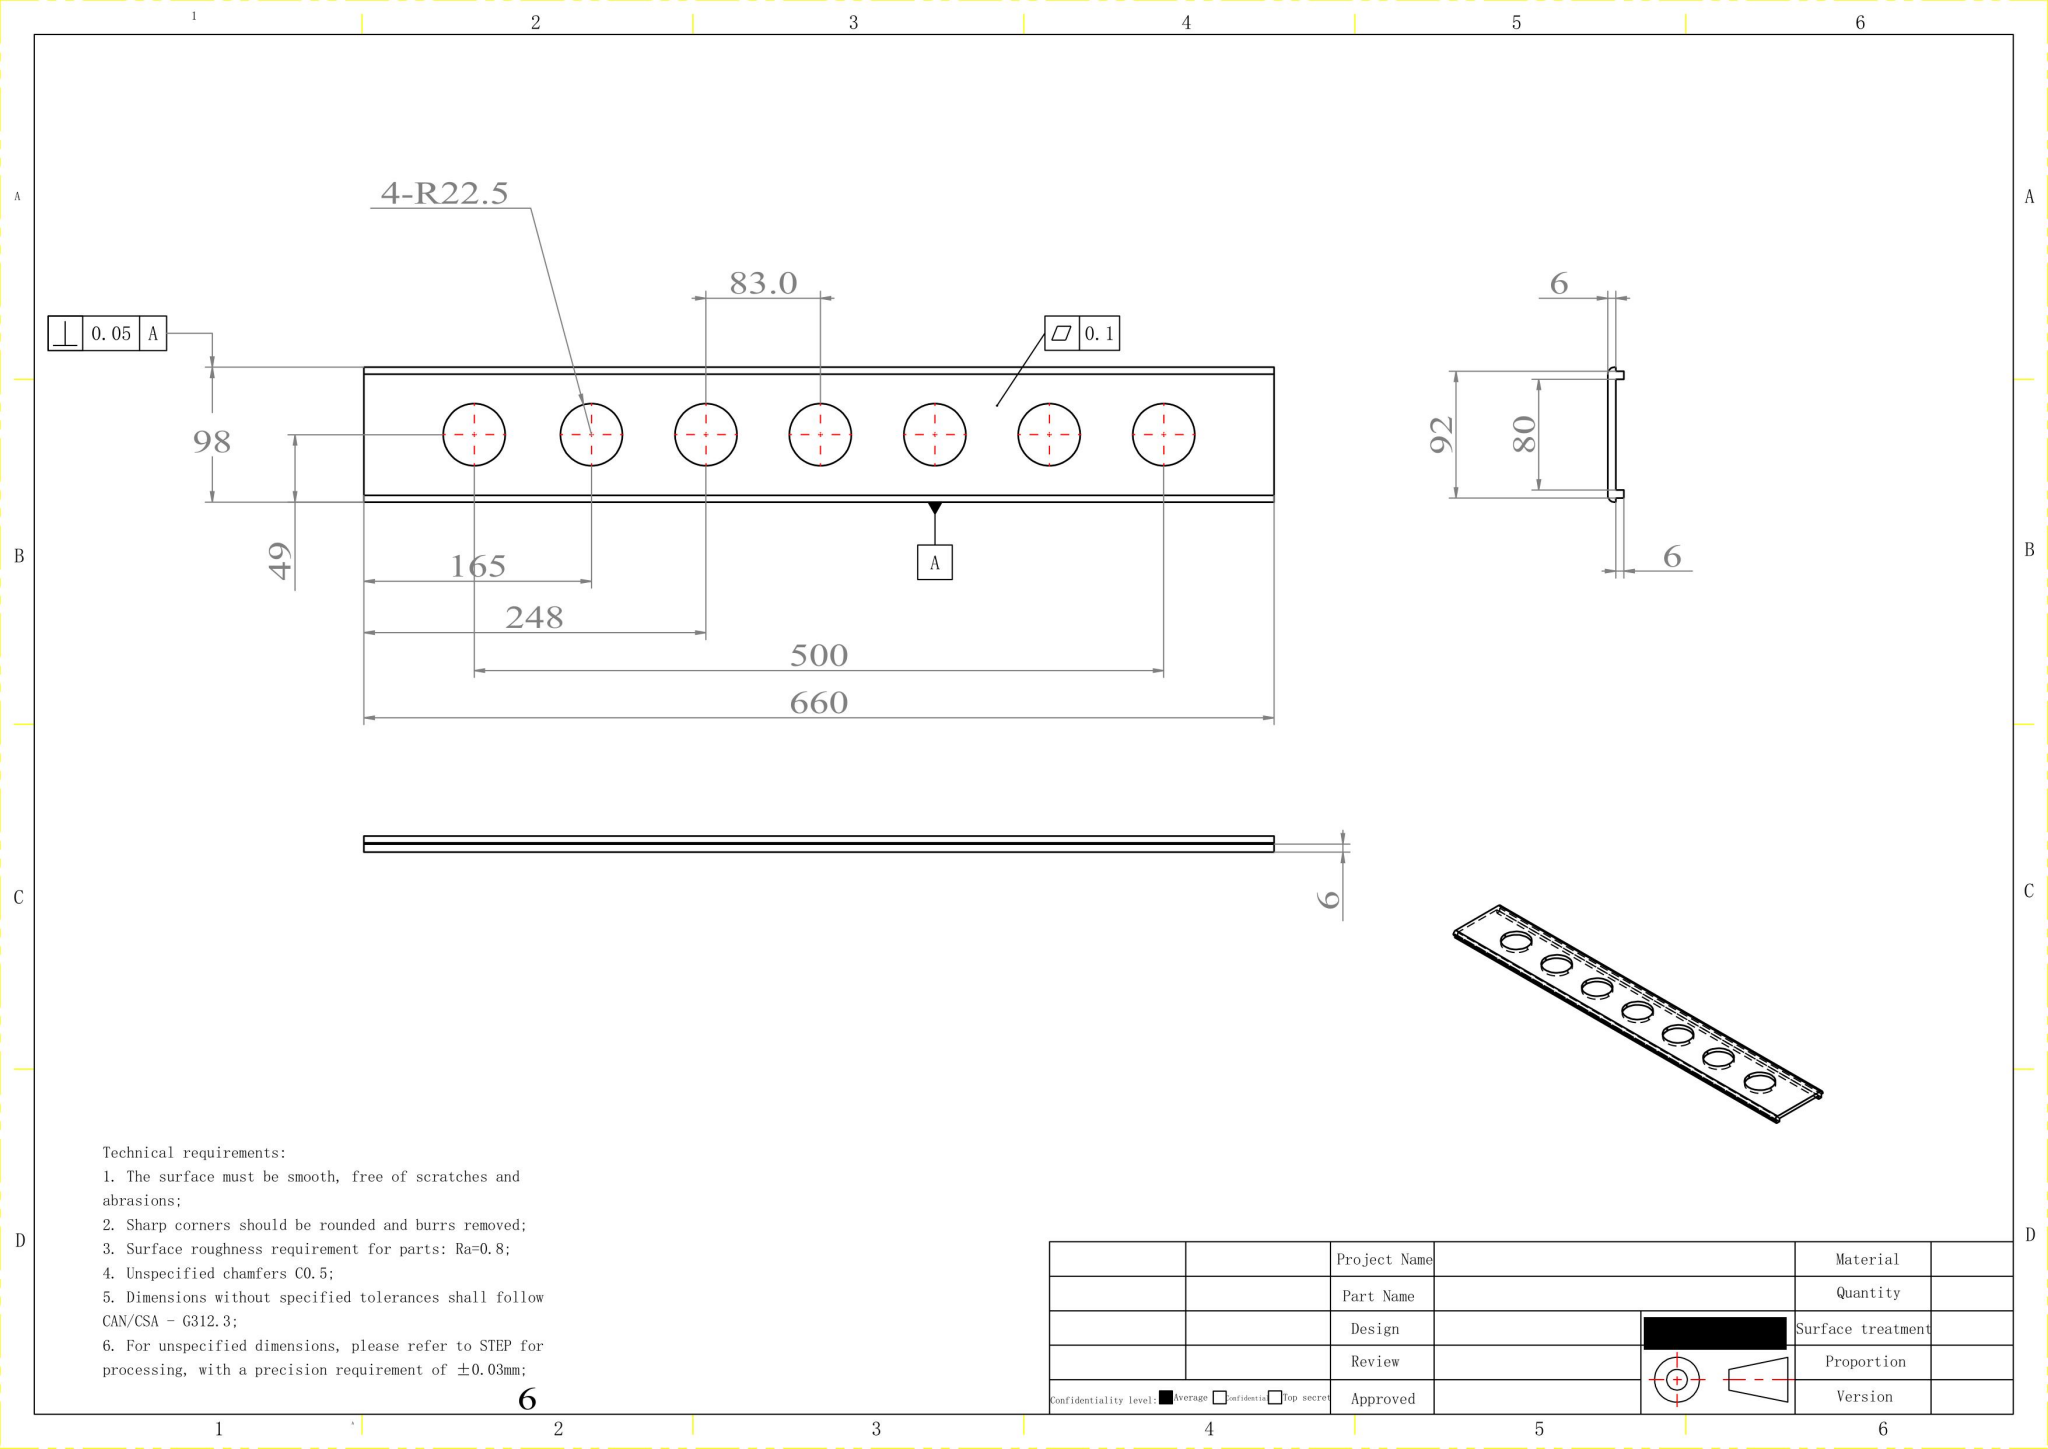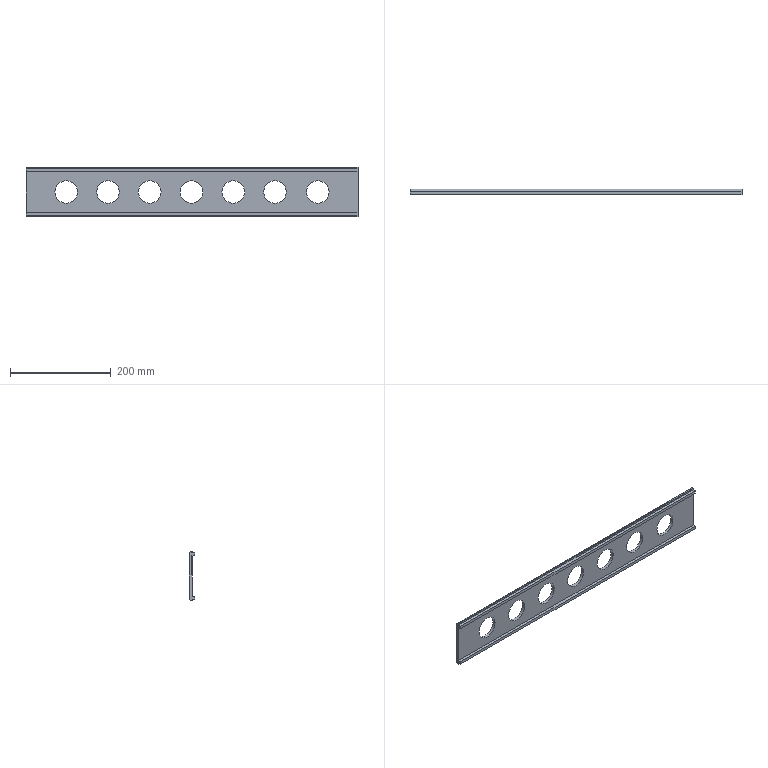Part | SolidWorks | mm | 1 solid | 30 faces | box 660 x 11.68 x 97.82 mm | volume 349958 mm3 | cylinder 16 | plane 14 | commonest cylinder face diameters 45 x14 10 x2
STEP:
#1=CARTESIAN_POINT('',(-165.31,-9.,-30.01));
#2=VERTEX_POINT('',#1);
#3=CARTESIAN_POINT('',(-825.31,-9.,-30.01));
#4=VERTEX_POINT('',#3);
#5=CARTESIAN_POINT('',(-165.31,-9.,-30.01));
#6=DIRECTION('',(-1.,0.,0.));
#7=VECTOR('',#6,1000.);
#8=LINE('',#5,#7);
#9=EDGE_CURVE('',#2,#4,#8,.T.);
#10=ORIENTED_EDGE('',*,*,#9,.F.);
#11=CARTESIAN_POINT('',(-165.31,-9.84,-30.01));
#12=VERTEX_POINT('',#11);
#13=CARTESIAN_POINT('',(-165.31,-9.84,-30.01));
#14=DIRECTION('',(0.,1.,-0.));
#15=VECTOR('',#14,1000.);
#16=LINE('',#13,#15);
#17=EDGE_CURVE('',#12,#2,#16,.T.);
#18=ORIENTED_EDGE('',*,*,#17,.F.);
#19=CARTESIAN_POINT('',(-825.31,-9.84,-30.01));
#20=VERTEX_POINT('',#19);
#21=CARTESIAN_POINT('',(-825.31,-9.84,-30.01));
#22=DIRECTION('',(1.,0.,0.));
#23=VECTOR('',#22,1000.);
#24=LINE('',#21,#23);
#25=EDGE_CURVE('',#20,#12,#24,.T.);
#26=ORIENTED_EDGE('',*,*,#25,.F.);
#27=CARTESIAN_POINT('',(-825.31,-9.,-30.01));
#28=DIRECTION('',(0.,-1.,0.));
#29=VECTOR('',#28,1000.);
#30=LINE('',#27,#29);
#31=EDGE_CURVE('',#4,#20,#30,.T.);
#32=ORIENTED_EDGE('',*,*,#31,.F.);
#33=EDGE_LOOP('',(#10,#18,#26,#32));
#34=FACE_OUTER_BOUND('',#33,.T.);
#35=CARTESIAN_POINT('',(-495.31,-9.84,-30.01));
#36=DIRECTION('',(0.,0.,-1.));
#37=DIRECTION('',(0.,-1.,0.));
#38=AXIS2_PLACEMENT_3D('',#35,#36,#37);
#39=PLANE('',#38);
#40=ADVANCED_FACE('',(#34),#39,.T.);
#41=CARTESIAN_POINT('',(-825.31,-4.,62.81));
#42=VERTEX_POINT('',#41);
#43=CARTESIAN_POINT('',(-825.31,-9.,67.81));
#44=VERTEX_POINT('',#43);
#45=CARTESIAN_POINT('',(-825.31,-9.,62.81));
#46=DIRECTION('',(1.,0.,0.));
#47=DIRECTION('',(-0.,1.,-0.));
#48=AXIS2_PLACEMENT_3D('',#45,#46,#47);
#49=CIRCLE('',#48,5.);
#50=EDGE_CURVE('',#42,#44,#49,.T.);
#51=ORIENTED_EDGE('',*,*,#50,.F.);
#52=CARTESIAN_POINT('',(-825.31,-4.,-25.01));
#53=VERTEX_POINT('',#52);
#54=CARTESIAN_POINT('',(-825.31,-4.,-25.01));
#55=DIRECTION('',(0.,0.,1.));
#56=VECTOR('',#55,1000.);
#57=LINE('',#54,#56);
#58=EDGE_CURVE('',#53,#42,#57,.T.);
#59=ORIENTED_EDGE('',*,*,#58,.F.);
#60=CARTESIAN_POINT('',(-825.31,-9.,-25.01));
#61=DIRECTION('',(1.,0.,-0.));
#62=DIRECTION('',(-0.,0.,-1.));
#63=AXIS2_PLACEMENT_3D('',#60,#61,#62);
#64=CIRCLE('',#63,5.);
#65=EDGE_CURVE('',#4,#53,#64,.T.);
#66=ORIENTED_EDGE('',*,*,#65,.F.);
#67=ORIENTED_EDGE('',*,*,#31,.T.);
#68=CARTESIAN_POINT('',(-825.31,-9.84,-27.09));
#69=VERTEX_POINT('',#68);
#70=CARTESIAN_POINT('',(-825.31,-9.84,-27.09));
#71=DIRECTION('',(0.,0.,-1.));
#72=VECTOR('',#71,1000.);
#73=LINE('',#70,#72);
#74=EDGE_CURVE('',#69,#20,#73,.T.);
#75=ORIENTED_EDGE('',*,*,#74,.F.);
#76=CARTESIAN_POINT('',(-825.31,-15.68,-27.09));
#77=VERTEX_POINT('',#76);
#78=CARTESIAN_POINT('',(-825.31,-15.68,-27.09));
#79=DIRECTION('',(0.,1.,0.));
#80=VECTOR('',#79,1000.);
#81=LINE('',#78,#80);
#82=EDGE_CURVE('',#77,#69,#81,.T.);
#83=ORIENTED_EDGE('',*,*,#82,.F.);
#84=CARTESIAN_POINT('',(-825.31,-15.68,-21.25));
#85=VERTEX_POINT('',#84);
#86=CARTESIAN_POINT('',(-825.31,-15.68,-21.25));
#87=DIRECTION('',(0.,0.,-1.));
#88=VECTOR('',#87,1000.);
#89=LINE('',#86,#88);
#90=EDGE_CURVE('',#85,#77,#89,.T.);
#91=ORIENTED_EDGE('',*,*,#90,.F.);
#92=CARTESIAN_POINT('',(-825.31,-9.84,-21.25));
#93=VERTEX_POINT('',#92);
#94=CARTESIAN_POINT('',(-825.31,-9.84,-21.25));
#95=DIRECTION('',(0.,-1.,0.));
#96=VECTOR('',#95,1000.);
#97=LINE('',#94,#96);
#98=EDGE_CURVE('',#93,#85,#97,.T.);
#99=ORIENTED_EDGE('',*,*,#98,.F.);
#100=CARTESIAN_POINT('',(-825.31,-9.84,59.05));
#101=VERTEX_POINT('',#100);
#102=CARTESIAN_POINT('',(-825.31,-9.84,59.05));
#103=DIRECTION('',(0.,0.,-1.));
#104=VECTOR('',#103,1000.);
#105=LINE('',#102,#104);
#106=EDGE_CURVE('',#101,#93,#105,.T.);
#107=ORIENTED_EDGE('',*,*,#106,.F.);
#108=CARTESIAN_POINT('',(-825.31,-15.68,59.05));
#109=VERTEX_POINT('',#108);
#110=CARTESIAN_POINT('',(-825.31,-15.68,59.05));
#111=DIRECTION('',(0.,1.,0.));
#112=VECTOR('',#111,1000.);
#113=LINE('',#110,#112);
#114=EDGE_CURVE('',#109,#101,#113,.T.);
#115=ORIENTED_EDGE('',*,*,#114,.F.);
#116=CARTESIAN_POINT('',(-825.31,-15.68,64.89));
#117=VERTEX_POINT('',#116);
#118=CARTESIAN_POINT('',(-825.31,-15.68,64.89));
#119=DIRECTION('',(0.,0.,-1.));
#120=VECTOR('',#119,1000.);
#121=LINE('',#118,#120);
#122=EDGE_CURVE('',#117,#109,#121,.T.);
#123=ORIENTED_EDGE('',*,*,#122,.F.);
#124=CARTESIAN_POINT('',(-825.31,-9.84,64.89));
#125=VERTEX_POINT('',#124);
#126=CARTESIAN_POINT('',(-825.31,-9.84,64.89));
#127=DIRECTION('',(0.,-1.,0.));
#128=VECTOR('',#127,1000.);
#129=LINE('',#126,#128);
#130=EDGE_CURVE('',#125,#117,#129,.T.);
#131=ORIENTED_EDGE('',*,*,#130,.F.);
#132=CARTESIAN_POINT('',(-825.31,-9.84,67.81));
#133=VERTEX_POINT('',#132);
#134=CARTESIAN_POINT('',(-825.31,-9.84,67.81));
#135=DIRECTION('',(0.,0.,-1.));
#136=VECTOR('',#135,1000.);
#137=LINE('',#134,#136);
#138=EDGE_CURVE('',#133,#125,#137,.T.);
#139=ORIENTED_EDGE('',*,*,#138,.F.);
#140=CARTESIAN_POINT('',(-825.31,-9.,67.81));
#141=DIRECTION('',(0.,-1.,0.));
#142=VECTOR('',#141,1000.);
#143=LINE('',#140,#142);
#144=EDGE_CURVE('',#44,#133,#143,.T.);
#145=ORIENTED_EDGE('',*,*,#144,.F.);
#146=EDGE_LOOP('',(#51,#59,#66,#67,#75,#83,#91,#99,#107,#115,#123,#131,#139,#145));
#147=FACE_OUTER_BOUND('',#146,.T.);
#148=CARTESIAN_POINT('',(-825.31,-4.,-35.85));
#149=DIRECTION('',(-1.,0.,0.));
#150=DIRECTION('',(0.,0.,1.));
#151=AXIS2_PLACEMENT_3D('',#148,#149,#150);
#152=PLANE('',#151);
#153=ADVANCED_FACE('',(#147),#152,.T.);
#154=CARTESIAN_POINT('',(-165.31,-9.84,-21.25));
#155=VERTEX_POINT('',#154);
#156=CARTESIAN_POINT('',(-165.31,-15.68,-21.25));
#157=VERTEX_POINT('',#156);
#158=CARTESIAN_POINT('',(-165.31,-9.84,-21.25));
#159=DIRECTION('',(0.,-1.,0.));
#160=VECTOR('',#159,1000.);
#161=LINE('',#158,#160);
#162=EDGE_CURVE('',#155,#157,#161,.T.);
#163=ORIENTED_EDGE('',*,*,#162,.F.);
#164=CARTESIAN_POINT('',(-825.31,-9.84,-21.25));
#165=DIRECTION('',(1.,0.,0.));
#166=VECTOR('',#165,1000.);
#167=LINE('',#164,#166);
#168=EDGE_CURVE('',#93,#155,#167,.T.);
#169=ORIENTED_EDGE('',*,*,#168,.F.);
#170=ORIENTED_EDGE('',*,*,#98,.T.);
#171=CARTESIAN_POINT('',(-165.31,-15.68,-21.25));
#172=DIRECTION('',(-1.,0.,0.));
#173=VECTOR('',#172,1000.);
#174=LINE('',#171,#173);
#175=EDGE_CURVE('',#157,#85,#174,.T.);
#176=ORIENTED_EDGE('',*,*,#175,.F.);
#177=EDGE_LOOP('',(#163,#169,#170,#176));
#178=FACE_OUTER_BOUND('',#177,.T.);
#179=CARTESIAN_POINT('',(-825.31,-9.84,-21.25));
#180=DIRECTION('',(0.,0.,1.));
#181=DIRECTION('',(0.,-1.,0.));
#182=AXIS2_PLACEMENT_3D('',#179,#180,#181);
#183=PLANE('',#182);
#184=ADVANCED_FACE('',(#178),#183,.T.);
#185=CARTESIAN_POINT('',(-165.31,-9.84,-27.09));
#186=VERTEX_POINT('',#185);
#187=CARTESIAN_POINT('',(-165.31,-9.84,-27.09));
#188=DIRECTION('',(0.,0.,-1.));
#189=VECTOR('',#188,1000.);
#190=LINE('',#187,#189);
#191=EDGE_CURVE('',#186,#12,#190,.T.);
#192=ORIENTED_EDGE('',*,*,#191,.F.);
#193=CARTESIAN_POINT('',(-825.31,-9.84,-27.09));
#194=DIRECTION('',(1.,0.,0.));
#195=VECTOR('',#194,1000.);
#196=LINE('',#193,#195);
#197=EDGE_CURVE('',#69,#186,#196,.T.);
#198=ORIENTED_EDGE('',*,*,#197,.F.);
#199=ORIENTED_EDGE('',*,*,#74,.T.);
#200=ORIENTED_EDGE('',*,*,#25,.T.);
#201=EDGE_LOOP('',(#192,#198,#199,#200));
#202=FACE_OUTER_BOUND('',#201,.T.);
#203=CARTESIAN_POINT('',(-825.31,-9.84,-27.09));
#204=DIRECTION('',(0.,-1.,0.));
#205=DIRECTION('',(0.,0.,-1.));
#206=AXIS2_PLACEMENT_3D('',#203,#204,#205);
#207=PLANE('',#206);
#208=ADVANCED_FACE('',(#202),#207,.T.);
#209=CARTESIAN_POINT('',(-165.31,-15.68,-27.09));
#210=VERTEX_POINT('',#209);
#211=CARTESIAN_POINT('',(-165.31,-15.68,-27.09));
#212=DIRECTION('',(0.,1.,0.));
#213=VECTOR('',#212,1000.);
#214=LINE('',#211,#213);
#215=EDGE_CURVE('',#210,#186,#214,.T.);
#216=ORIENTED_EDGE('',*,*,#215,.F.);
#217=CARTESIAN_POINT('',(-825.31,-15.68,-27.09));
#218=DIRECTION('',(1.,0.,0.));
#219=VECTOR('',#218,1000.);
#220=LINE('',#217,#219);
#221=EDGE_CURVE('',#77,#210,#220,.T.);
#222=ORIENTED_EDGE('',*,*,#221,.F.);
#223=ORIENTED_EDGE('',*,*,#82,.T.);
#224=ORIENTED_EDGE('',*,*,#197,.T.);
#225=EDGE_LOOP('',(#216,#222,#223,#224));
#226=FACE_OUTER_BOUND('',#225,.T.);
#227=CARTESIAN_POINT('',(-825.31,-9.84,-27.09));
#228=DIRECTION('',(0.,0.,-1.));
#229=DIRECTION('',(0.,-1.,0.));
#230=AXIS2_PLACEMENT_3D('',#227,#228,#229);
#231=PLANE('',#230);
#232=ADVANCED_FACE('',(#226),#231,.T.);
#233=CARTESIAN_POINT('',(-165.31,-15.68,-21.25));
#234=DIRECTION('',(0.,0.,-1.));
#235=VECTOR('',#234,1000.);
#236=LINE('',#233,#235);
#237=EDGE_CURVE('',#157,#210,#236,.T.);
#238=ORIENTED_EDGE('',*,*,#237,.F.);
#239=ORIENTED_EDGE('',*,*,#175,.T.);
#240=ORIENTED_EDGE('',*,*,#90,.T.);
#241=ORIENTED_EDGE('',*,*,#221,.T.);
#242=EDGE_LOOP('',(#238,#239,#240,#241));
#243=FACE_OUTER_BOUND('',#242,.T.);
#244=CARTESIAN_POINT('',(-222.834,-15.68,18.9));
#245=DIRECTION('',(0.,-1.,0.));
#246=DIRECTION('',(0.,0.,-1.));
#247=AXIS2_PLACEMENT_3D('',#244,#245,#246);
#248=PLANE('',#247);
#249=ADVANCED_FACE('',(#243),#248,.T.);
#250=CARTESIAN_POINT('',(-165.31,-9.84,67.81));
#251=VERTEX_POINT('',#250);
#252=CARTESIAN_POINT('',(-165.31,-9.84,64.89));
#253=VERTEX_POINT('',#252);
#254=CARTESIAN_POINT('',(-165.31,-9.84,67.81));
#255=DIRECTION('',(0.,0.,-1.));
#256=VECTOR('',#255,1000.);
#257=LINE('',#254,#256);
#258=EDGE_CURVE('',#251,#253,#257,.T.);
#259=ORIENTED_EDGE('',*,*,#258,.F.);
#260=CARTESIAN_POINT('',(-825.31,-9.84,67.81));
#261=DIRECTION('',(1.,0.,0.));
#262=VECTOR('',#261,1000.);
#263=LINE('',#260,#262);
#264=EDGE_CURVE('',#133,#251,#263,.T.);
#265=ORIENTED_EDGE('',*,*,#264,.F.);
#266=ORIENTED_EDGE('',*,*,#138,.T.);
#267=CARTESIAN_POINT('',(-165.31,-9.84,64.89));
#268=DIRECTION('',(-1.,0.,0.));
#269=VECTOR('',#268,1000.);
#270=LINE('',#267,#269);
#271=EDGE_CURVE('',#253,#125,#270,.T.);
#272=ORIENTED_EDGE('',*,*,#271,.F.);
#273=EDGE_LOOP('',(#259,#265,#266,#272));
#274=FACE_OUTER_BOUND('',#273,.T.);
#275=CARTESIAN_POINT('',(-825.31,-9.84,67.81));
#276=DIRECTION('',(0.,-1.,0.));
#277=DIRECTION('',(0.,0.,-1.));
#278=AXIS2_PLACEMENT_3D('',#275,#276,#277);
#279=PLANE('',#278);
#280=ADVANCED_FACE('',(#274),#279,.T.);
#281=CARTESIAN_POINT('',(-165.31,-15.68,64.89));
#282=VERTEX_POINT('',#281);
#283=CARTESIAN_POINT('',(-165.31,-9.84,64.89));
#284=DIRECTION('',(0.,-1.,0.));
#285=VECTOR('',#284,1000.);
#286=LINE('',#283,#285);
#287=EDGE_CURVE('',#253,#282,#286,.T.);
#288=ORIENTED_EDGE('',*,*,#287,.F.);
#289=ORIENTED_EDGE('',*,*,#271,.T.);
#290=ORIENTED_EDGE('',*,*,#130,.T.);
#291=CARTESIAN_POINT('',(-165.31,-15.68,64.89));
#292=DIRECTION('',(-1.,0.,0.));
#293=VECTOR('',#292,1000.);
#294=LINE('',#291,#293);
#295=EDGE_CURVE('',#282,#117,#294,.T.);
#296=ORIENTED_EDGE('',*,*,#295,.F.);
#297=EDGE_LOOP('',(#288,#289,#290,#296));
#298=FACE_OUTER_BOUND('',#297,.T.);
#299=CARTESIAN_POINT('',(-825.31,-9.84,64.89));
#300=DIRECTION('',(0.,0.,1.));
#301=DIRECTION('',(1.,0.,0.));
#302=AXIS2_PLACEMENT_3D('',#299,#300,#301);
#303=PLANE('',#302);
#304=ADVANCED_FACE('',(#298),#303,.T.);
#305=CARTESIAN_POINT('',(-165.31,-15.68,59.05));
#306=VERTEX_POINT('',#305);
#307=CARTESIAN_POINT('',(-165.31,-15.68,64.89));
#308=DIRECTION('',(0.,0.,-1.));
#309=VECTOR('',#308,1000.);
#310=LINE('',#307,#309);
#311=EDGE_CURVE('',#282,#306,#310,.T.);
#312=ORIENTED_EDGE('',*,*,#311,.F.);
#313=ORIENTED_EDGE('',*,*,#295,.T.);
#314=ORIENTED_EDGE('',*,*,#122,.T.);
#315=CARTESIAN_POINT('',(-165.31,-15.68,59.05));
#316=DIRECTION('',(-1.,0.,0.));
#317=VECTOR('',#316,1000.);
#318=LINE('',#315,#317);
#319=EDGE_CURVE('',#306,#109,#318,.T.);
#320=ORIENTED_EDGE('',*,*,#319,.F.);
#321=EDGE_LOOP('',(#312,#313,#314,#320));
#322=FACE_OUTER_BOUND('',#321,.T.);
#323=CARTESIAN_POINT('',(-222.834,-15.68,18.9));
#324=DIRECTION('',(0.,-1.,0.));
#325=DIRECTION('',(0.,0.,-1.));
#326=AXIS2_PLACEMENT_3D('',#323,#324,#325);
#327=PLANE('',#326);
#328=ADVANCED_FACE('',(#322),#327,.T.);
#329=CARTESIAN_POINT('',(-165.31,-9.84,59.05));
#330=VERTEX_POINT('',#329);
#331=CARTESIAN_POINT('',(-165.31,-15.68,59.05));
#332=DIRECTION('',(0.,1.,0.));
#333=VECTOR('',#332,1000.);
#334=LINE('',#331,#333);
#335=EDGE_CURVE('',#306,#330,#334,.T.);
#336=ORIENTED_EDGE('',*,*,#335,.F.);
#337=ORIENTED_EDGE('',*,*,#319,.T.);
#338=ORIENTED_EDGE('',*,*,#114,.T.);
#339=CARTESIAN_POINT('',(-165.31,-9.84,59.05));
#340=DIRECTION('',(-1.,0.,0.));
#341=VECTOR('',#340,1000.);
#342=LINE('',#339,#341);
#343=EDGE_CURVE('',#330,#101,#342,.T.);
#344=ORIENTED_EDGE('',*,*,#343,.F.);
#345=EDGE_LOOP('',(#336,#337,#338,#344));
#346=FACE_OUTER_BOUND('',#345,.T.);
#347=CARTESIAN_POINT('',(-825.31,-9.84,59.05));
#348=DIRECTION('',(0.,0.,-1.));
#349=DIRECTION('',(0.,-1.,0.));
#350=AXIS2_PLACEMENT_3D('',#347,#348,#349);
#351=PLANE('',#350);
#352=ADVANCED_FACE('',(#346),#351,.T.);
#353=CARTESIAN_POINT('',(-435.81,-9.84,18.9));
#354=VERTEX_POINT('',#353);
#355=CARTESIAN_POINT('',(-390.81,-9.84,18.9));
#356=VERTEX_POINT('',#355);
#357=CARTESIAN_POINT('',(-413.31,-9.84,18.9));
#358=DIRECTION('',(-0.,-1.,0.));
#359=DIRECTION('',(-1.,0.,-0.));
#360=AXIS2_PLACEMENT_3D('',#357,#358,#359);
#361=CIRCLE('',#360,22.5);
#362=EDGE_CURVE('',#354,#356,#361,.T.);
#363=ORIENTED_EDGE('',*,*,#362,.F.);
#364=CARTESIAN_POINT('',(-413.31,-9.84,18.9));
#365=DIRECTION('',(0.,-1.,-0.));
#366=DIRECTION('',(1.,0.,0.));
#367=AXIS2_PLACEMENT_3D('',#364,#365,#366);
#368=CIRCLE('',#367,22.5);
#369=EDGE_CURVE('',#356,#354,#368,.T.);
#370=ORIENTED_EDGE('',*,*,#369,.F.);
#371=EDGE_LOOP('',(#363,#370));
#372=FACE_BOUND('',#371,.T.);
#373=CARTESIAN_POINT('',(-767.81,-9.84,18.9));
#374=VERTEX_POINT('',#373);
#375=CARTESIAN_POINT('',(-722.81,-9.84,18.9));
#376=VERTEX_POINT('',#375);
#377=CARTESIAN_POINT('',(-745.31,-9.84,18.9));
#378=DIRECTION('',(0.,-1.,-0.));
#379=DIRECTION('',(-1.,-0.,0.));
#380=AXIS2_PLACEMENT_3D('',#377,#378,#379);
#381=CIRCLE('',#380,22.5);
#382=EDGE_CURVE('',#374,#376,#381,.T.);
#383=ORIENTED_EDGE('',*,*,#382,.F.);
#384=CARTESIAN_POINT('',(-745.31,-9.84,18.9));
#385=DIRECTION('',(0.,-1.,-0.));
#386=DIRECTION('',(1.,0.,0.));
#387=AXIS2_PLACEMENT_3D('',#384,#385,#386);
#388=CIRCLE('',#387,22.5);
#389=EDGE_CURVE('',#376,#374,#388,.T.);
#390=ORIENTED_EDGE('',*,*,#389,.F.);
#391=EDGE_LOOP('',(#383,#390));
#392=FACE_BOUND('',#391,.T.);
#393=CARTESIAN_POINT('',(-518.81,-9.84,18.9));
#394=VERTEX_POINT('',#393);
#395=CARTESIAN_POINT('',(-473.81,-9.84,18.9));
#396=VERTEX_POINT('',#395);
#397=CARTESIAN_POINT('',(-496.31,-9.84,18.9));
#398=DIRECTION('',(-0.,-1.,-0.));
#399=DIRECTION('',(-1.,0.,0.));
#400=AXIS2_PLACEMENT_3D('',#397,#398,#399);
#401=CIRCLE('',#400,22.5);
#402=EDGE_CURVE('',#394,#396,#401,.T.);
#403=ORIENTED_EDGE('',*,*,#402,.F.);
#404=CARTESIAN_POINT('',(-496.31,-9.84,18.9));
#405=DIRECTION('',(0.,-1.,-0.));
#406=DIRECTION('',(1.,0.,0.));
#407=AXIS2_PLACEMENT_3D('',#404,#405,#406);
#408=CIRCLE('',#407,22.5);
#409=EDGE_CURVE('',#396,#394,#408,.T.);
#410=ORIENTED_EDGE('',*,*,#409,.F.);
#411=EDGE_LOOP('',(#403,#410));
#412=FACE_BOUND('',#411,.T.);
#413=CARTESIAN_POINT('',(-267.81,-9.84,18.9));
#414=VERTEX_POINT('',#413);
#415=CARTESIAN_POINT('',(-222.81,-9.84,18.9));
#416=VERTEX_POINT('',#415);
#417=CARTESIAN_POINT('',(-245.31,-9.84,18.9));
#418=DIRECTION('',(0.,-1.,-0.));
#419=DIRECTION('',(-1.,0.,-0.));
#420=AXIS2_PLACEMENT_3D('',#417,#418,#419);
#421=CIRCLE('',#420,22.5);
#422=EDGE_CURVE('',#414,#416,#421,.T.);
#423=ORIENTED_EDGE('',*,*,#422,.F.);
#424=CARTESIAN_POINT('',(-245.31,-9.84,18.9));
#425=DIRECTION('',(-0.,-1.,-0.));
#426=DIRECTION('',(1.,0.,-0.));
#427=AXIS2_PLACEMENT_3D('',#424,#425,#426);
#428=CIRCLE('',#427,22.5);
#429=EDGE_CURVE('',#416,#414,#428,.T.);
#430=ORIENTED_EDGE('',*,*,#429,.F.);
#431=EDGE_LOOP('',(#423,#430));
#432=FACE_BOUND('',#431,.T.);
#433=CARTESIAN_POINT('',(-684.81,-9.84,18.9));
#434=VERTEX_POINT('',#433);
#435=CARTESIAN_POINT('',(-639.81,-9.84,18.9));
#436=VERTEX_POINT('',#435);
#437=CARTESIAN_POINT('',(-662.31,-9.84,18.9));
#438=DIRECTION('',(0.,-1.,-0.));
#439=DIRECTION('',(-1.,-0.,0.));
#440=AXIS2_PLACEMENT_3D('',#437,#438,#439);
#441=CIRCLE('',#440,22.5);
#442=EDGE_CURVE('',#434,#436,#441,.T.);
#443=ORIENTED_EDGE('',*,*,#442,.F.);
#444=CARTESIAN_POINT('',(-662.31,-9.84,18.9));
#445=DIRECTION('',(0.,-1.,-0.));
#446=DIRECTION('',(1.,0.,0.));
#447=AXIS2_PLACEMENT_3D('',#444,#445,#446);
#448=CIRCLE('',#447,22.5);
#449=EDGE_CURVE('',#436,#434,#448,.T.);
#450=ORIENTED_EDGE('',*,*,#449,.F.);
#451=EDGE_LOOP('',(#443,#450));
#452=FACE_BOUND('',#451,.T.);
#453=CARTESIAN_POINT('',(-601.81,-9.84,18.9));
#454=VERTEX_POINT('',#453);
#455=CARTESIAN_POINT('',(-556.81,-9.84,18.9));
#456=VERTEX_POINT('',#455);
#457=CARTESIAN_POINT('',(-579.31,-9.84,18.9));
#458=DIRECTION('',(0.,-1.,-0.));
#459=DIRECTION('',(-1.,-0.,0.));
#460=AXIS2_PLACEMENT_3D('',#457,#458,#459);
#461=CIRCLE('',#460,22.5);
#462=EDGE_CURVE('',#454,#456,#461,.T.);
#463=ORIENTED_EDGE('',*,*,#462,.F.);
#464=CARTESIAN_POINT('',(-579.31,-9.84,18.9));
#465=DIRECTION('',(0.,-1.,-0.));
#466=DIRECTION('',(1.,0.,0.));
#467=AXIS2_PLACEMENT_3D('',#464,#465,#466);
#468=CIRCLE('',#467,22.5);
#469=EDGE_CURVE('',#456,#454,#468,.T.);
#470=ORIENTED_EDGE('',*,*,#469,.F.);
#471=EDGE_LOOP('',(#463,#470));
#472=FACE_BOUND('',#471,.T.);
#473=CARTESIAN_POINT('',(-352.81,-9.84,18.9));
#474=VERTEX_POINT('',#473);
#475=CARTESIAN_POINT('',(-307.81,-9.84,18.9));
#476=VERTEX_POINT('',#475);
#477=CARTESIAN_POINT('',(-330.31,-9.84,18.9));
#478=DIRECTION('',(0.,-1.,-0.));
#479=DIRECTION('',(-1.,-0.,0.));
#480=AXIS2_PLACEMENT_3D('',#477,#478,#479);
#481=CIRCLE('',#480,22.5);
#482=EDGE_CURVE('',#474,#476,#481,.T.);
#483=ORIENTED_EDGE('',*,*,#482,.F.);
#484=CARTESIAN_POINT('',(-330.31,-9.84,18.9));
#485=DIRECTION('',(0.,-1.,-0.));
#486=DIRECTION('',(1.,0.,0.));
#487=AXIS2_PLACEMENT_3D('',#484,#485,#486);
#488=CIRCLE('',#487,22.5);
#489=EDGE_CURVE('',#476,#474,#488,.T.);
#490=ORIENTED_EDGE('',*,*,#489,.F.);
#491=EDGE_LOOP('',(#483,#490));
#492=FACE_BOUND('',#491,.T.);
#493=CARTESIAN_POINT('',(-165.31,-9.84,59.05));
#494=DIRECTION('',(0.,0.,-1.));
#495=VECTOR('',#494,1000.);
#496=LINE('',#493,#495);
#497=EDGE_CURVE('',#330,#155,#496,.T.);
#498=ORIENTED_EDGE('',*,*,#497,.F.);
#499=ORIENTED_EDGE('',*,*,#343,.T.);
#500=ORIENTED_EDGE('',*,*,#106,.T.);
#501=ORIENTED_EDGE('',*,*,#168,.T.);
#502=EDGE_LOOP('',(#498,#499,#500,#501));
#503=FACE_OUTER_BOUND('',#502,.T.);
#504=CARTESIAN_POINT('',(-825.31,-9.84,59.05));
#505=DIRECTION('',(0.,-1.,0.));
#506=DIRECTION('',(0.,0.,-1.));
#507=AXIS2_PLACEMENT_3D('',#504,#505,#506);
#508=PLANE('',#507);
#509=ADVANCED_FACE('',(#372,#392,#412,#432,#452,#472,#492,#503),#508,.T.);
#510=CARTESIAN_POINT('',(-352.81,-4.,18.9));
#511=VERTEX_POINT('',#510);
#512=CARTESIAN_POINT('',(-307.81,-4.,18.9));
#513=VERTEX_POINT('',#512);
#514=CARTESIAN_POINT('',(-330.31,-4.,18.9));
#515=DIRECTION('',(0.,-1.,0.));
#516=DIRECTION('',(-1.,0.,-0.));
#517=AXIS2_PLACEMENT_3D('',#514,#515,#516);
#518=CIRCLE('',#517,22.5);
#519=EDGE_CURVE('',#511,#513,#518,.T.);
#520=ORIENTED_EDGE('',*,*,#519,.F.);
#521=CARTESIAN_POINT('',(-352.81,-9.84,18.9));
#522=DIRECTION('',(0.,1.,0.));
#523=VECTOR('',#522,1000.);
#524=LINE('',#521,#523);
#525=EDGE_CURVE('',#474,#511,#524,.T.);
#526=ORIENTED_EDGE('',*,*,#525,.F.);
#527=ORIENTED_EDGE('',*,*,#482,.T.);
#528=CARTESIAN_POINT('',(-307.81,-4.,18.9));
#529=DIRECTION('',(0.,-1.,0.));
#530=VECTOR('',#529,1000.);
#531=LINE('',#528,#530);
#532=EDGE_CURVE('',#513,#476,#531,.T.);
#533=ORIENTED_EDGE('',*,*,#532,.F.);
#534=EDGE_LOOP('',(#520,#526,#527,#533));
#535=FACE_OUTER_BOUND('',#534,.T.);
#536=CARTESIAN_POINT('',(-330.31,-4.,18.9));
#537=DIRECTION('',(0.,-1.,-0.));
#538=DIRECTION('',(-1.,-0.,0.));
#539=AXIS2_PLACEMENT_3D('',#536,#537,#538);
#540=CYLINDRICAL_SURFACE('',#539,22.5);
#541=ADVANCED_FACE('',(#535),#540,.F.);
#542=ORIENTED_EDGE('',*,*,#532,.T.);
#543=ORIENTED_EDGE('',*,*,#489,.T.);
#544=ORIENTED_EDGE('',*,*,#525,.T.);
#545=CARTESIAN_POINT('',(-330.31,-4.,18.9));
#546=DIRECTION('',(0.,-1.,0.));
#547=DIRECTION('',(1.,0.,0.));
#548=AXIS2_PLACEMENT_3D('',#545,#546,#547);
#549=CIRCLE('',#548,22.5);
#550=EDGE_CURVE('',#513,#511,#549,.T.);
#551=ORIENTED_EDGE('',*,*,#550,.F.);
#552=EDGE_LOOP('',(#542,#543,#544,#551));
#553=FACE_OUTER_BOUND('',#552,.T.);
#554=CARTESIAN_POINT('',(-330.31,-4.,18.9));
#555=DIRECTION('',(0.,-1.,-0.));
#556=DIRECTION('',(-1.,-0.,0.));
#557=AXIS2_PLACEMENT_3D('',#554,#555,#556);
#558=CYLINDRICAL_SURFACE('',#557,22.5);
#559=ADVANCED_FACE('',(#553),#558,.F.);
#560=CARTESIAN_POINT('',(-601.81,-4.,18.9));
#561=VERTEX_POINT('',#560);
#562=CARTESIAN_POINT('',(-556.81,-4.,18.9));
#563=VERTEX_POINT('',#562);
#564=CARTESIAN_POINT('',(-579.31,-4.,18.9));
#565=DIRECTION('',(0.,-1.,0.));
#566=DIRECTION('',(-1.,0.,0.));
#567=AXIS2_PLACEMENT_3D('',#564,#565,#566);
#568=CIRCLE('',#567,22.5);
#569=EDGE_CURVE('',#561,#563,#568,.T.);
#570=ORIENTED_EDGE('',*,*,#569,.F.);
#571=CARTESIAN_POINT('',(-601.81,-9.84,18.9));
#572=DIRECTION('',(-0.,1.,0.));
#573=VECTOR('',#572,1000.);
#574=LINE('',#571,#573);
#575=EDGE_CURVE('',#454,#561,#574,.T.);
#576=ORIENTED_EDGE('',*,*,#575,.F.);
#577=ORIENTED_EDGE('',*,*,#462,.T.);
#578=CARTESIAN_POINT('',(-556.81,-4.,18.9));
#579=DIRECTION('',(0.,-1.,0.));
#580=VECTOR('',#579,1000.);
#581=LINE('',#578,#580);
#582=EDGE_CURVE('',#563,#456,#581,.T.);
#583=ORIENTED_EDGE('',*,*,#582,.F.);
#584=EDGE_LOOP('',(#570,#576,#577,#583));
#585=FACE_OUTER_BOUND('',#584,.T.);
#586=CARTESIAN_POINT('',(-579.31,-4.,18.9));
#587=DIRECTION('',(0.,-1.,-0.));
#588=DIRECTION('',(-1.,-0.,0.));
#589=AXIS2_PLACEMENT_3D('',#586,#587,#588);
#590=CYLINDRICAL_SURFACE('',#589,22.5);
#591=ADVANCED_FACE('',(#585),#590,.F.);
#592=ORIENTED_EDGE('',*,*,#582,.T.);
#593=ORIENTED_EDGE('',*,*,#469,.T.);
#594=ORIENTED_EDGE('',*,*,#575,.T.);
#595=CARTESIAN_POINT('',(-579.31,-4.,18.9));
#596=DIRECTION('',(0.,-1.,0.));
#597=DIRECTION('',(1.,0.,-0.));
#598=AXIS2_PLACEMENT_3D('',#595,#596,#597);
#599=CIRCLE('',#598,22.5);
#600=EDGE_CURVE('',#563,#561,#599,.T.);
#601=ORIENTED_EDGE('',*,*,#600,.F.);
#602=EDGE_LOOP('',(#592,#593,#594,#601));
#603=FACE_OUTER_BOUND('',#602,.T.);
#604=CARTESIAN_POINT('',(-579.31,-4.,18.9));
#605=DIRECTION('',(0.,-1.,-0.));
#606=DIRECTION('',(-1.,-0.,0.));
#607=AXIS2_PLACEMENT_3D('',#604,#605,#606);
#608=CYLINDRICAL_SURFACE('',#607,22.5);
#609=ADVANCED_FACE('',(#603),#608,.F.);
#610=CARTESIAN_POINT('',(-684.81,-4.,18.9));
#611=VERTEX_POINT('',#610);
#612=CARTESIAN_POINT('',(-639.81,-4.,18.9));
#613=VERTEX_POINT('',#612);
#614=CARTESIAN_POINT('',(-662.31,-4.,18.9));
#615=DIRECTION('',(0.,-1.,0.));
#616=DIRECTION('',(-1.,0.,-0.));
#617=AXIS2_PLACEMENT_3D('',#614,#615,#616);
#618=CIRCLE('',#617,22.5);
#619=EDGE_CURVE('',#611,#613,#618,.T.);
#620=ORIENTED_EDGE('',*,*,#619,.F.);
#621=CARTESIAN_POINT('',(-684.81,-9.84,18.9));
#622=DIRECTION('',(0.,1.,0.));
#623=VECTOR('',#622,1000.);
#624=LINE('',#621,#623);
#625=EDGE_CURVE('',#434,#611,#624,.T.);
#626=ORIENTED_EDGE('',*,*,#625,.F.);
#627=ORIENTED_EDGE('',*,*,#442,.T.);
#628=CARTESIAN_POINT('',(-639.81,-4.,18.9));
#629=DIRECTION('',(0.,-1.,0.));
#630=VECTOR('',#629,1000.);
#631=LINE('',#628,#630);
#632=EDGE_CURVE('',#613,#436,#631,.T.);
#633=ORIENTED_EDGE('',*,*,#632,.F.);
#634=EDGE_LOOP('',(#620,#626,#627,#633));
#635=FACE_OUTER_BOUND('',#634,.T.);
#636=CARTESIAN_POINT('',(-662.31,-4.,18.9));
#637=DIRECTION('',(0.,-1.,-0.));
#638=DIRECTION('',(-1.,-0.,0.));
#639=AXIS2_PLACEMENT_3D('',#636,#637,#638);
#640=CYLINDRICAL_SURFACE('',#639,22.5);
#641=ADVANCED_FACE('',(#635),#640,.F.);
#642=ORIENTED_EDGE('',*,*,#632,.T.);
#643=ORIENTED_EDGE('',*,*,#449,.T.);
#644=ORIENTED_EDGE('',*,*,#625,.T.);
#645=CARTESIAN_POINT('',(-662.31,-4.,18.9));
#646=DIRECTION('',(0.,-1.,0.));
#647=DIRECTION('',(1.,0.,0.));
#648=AXIS2_PLACEMENT_3D('',#645,#646,#647);
#649=CIRCLE('',#648,22.5);
#650=EDGE_CURVE('',#613,#611,#649,.T.);
#651=ORIENTED_EDGE('',*,*,#650,.F.);
#652=EDGE_LOOP('',(#642,#643,#644,#651));
#653=FACE_OUTER_BOUND('',#652,.T.);
#654=CARTESIAN_POINT('',(-662.31,-4.,18.9));
#655=DIRECTION('',(0.,-1.,-0.));
#656=DIRECTION('',(-1.,-0.,0.));
#657=AXIS2_PLACEMENT_3D('',#654,#655,#656);
#658=CYLINDRICAL_SURFACE('',#657,22.5);
#659=ADVANCED_FACE('',(#653),#658,.F.);
#660=CARTESIAN_POINT('',(-267.81,-4.,18.9));
#661=VERTEX_POINT('',#660);
#662=CARTESIAN_POINT('',(-222.81,-4.,18.9));
#663=VERTEX_POINT('',#662);
#664=CARTESIAN_POINT('',(-245.31,-4.,18.9));
#665=DIRECTION('',(0.,-1.,0.));
#666=DIRECTION('',(-1.,0.,0.));
#667=AXIS2_PLACEMENT_3D('',#664,#665,#666);
#668=CIRCLE('',#667,22.5);
#669=EDGE_CURVE('',#661,#663,#668,.T.);
#670=ORIENTED_EDGE('',*,*,#669,.F.);
#671=CARTESIAN_POINT('',(-267.81,-9.84,18.9));
#672=DIRECTION('',(0.,1.,0.));
#673=VECTOR('',#672,1000.);
#674=LINE('',#671,#673);
#675=EDGE_CURVE('',#414,#661,#674,.T.);
#676=ORIENTED_EDGE('',*,*,#675,.F.);
#677=ORIENTED_EDGE('',*,*,#422,.T.);
#678=CARTESIAN_POINT('',(-222.81,-4.,18.9));
#679=DIRECTION('',(0.,-1.,0.));
#680=VECTOR('',#679,1000.);
#681=LINE('',#678,#680);
#682=EDGE_CURVE('',#663,#416,#681,.T.);
#683=ORIENTED_EDGE('',*,*,#682,.F.);
#684=EDGE_LOOP('',(#670,#676,#677,#683));
#685=FACE_OUTER_BOUND('',#684,.T.);
#686=CARTESIAN_POINT('',(-245.31,-4.,18.9));
#687=DIRECTION('',(0.,-1.,0.));
#688=DIRECTION('',(-1.,-0.,0.));
#689=AXIS2_PLACEMENT_3D('',#686,#687,#688);
#690=CYLINDRICAL_SURFACE('',#689,22.5);
#691=ADVANCED_FACE('',(#685),#690,.F.);
#692=ORIENTED_EDGE('',*,*,#682,.T.);
#693=ORIENTED_EDGE('',*,*,#429,.T.);
#694=ORIENTED_EDGE('',*,*,#675,.T.);
#695=CARTESIAN_POINT('',(-245.31,-4.,18.9));
#696=DIRECTION('',(0.,-1.,0.));
#697=DIRECTION('',(1.,0.,0.));
#698=AXIS2_PLACEMENT_3D('',#695,#696,#697);
#699=CIRCLE('',#698,22.5);
#700=EDGE_CURVE('',#663,#661,#699,.T.);
#701=ORIENTED_EDGE('',*,*,#700,.F.);
#702=EDGE_LOOP('',(#692,#693,#694,#701));
#703=FACE_OUTER_BOUND('',#702,.T.);
#704=CARTESIAN_POINT('',(-245.31,-4.,18.9));
#705=DIRECTION('',(0.,-1.,0.));
#706=DIRECTION('',(-1.,-0.,0.));
#707=AXIS2_PLACEMENT_3D('',#704,#705,#706);
#708=CYLINDRICAL_SURFACE('',#707,22.5);
#709=ADVANCED_FACE('',(#703),#708,.F.);
#710=CARTESIAN_POINT('',(-518.81,-4.,18.9));
#711=VERTEX_POINT('',#710);
#712=CARTESIAN_POINT('',(-473.81,-4.,18.9));
#713=VERTEX_POINT('',#712);
#714=CARTESIAN_POINT('',(-496.31,-4.,18.9));
#715=DIRECTION('',(0.,-1.,0.));
#716=DIRECTION('',(-1.,0.,-0.));
#717=AXIS2_PLACEMENT_3D('',#714,#715,#716);
#718=CIRCLE('',#717,22.5);
#719=EDGE_CURVE('',#711,#713,#718,.T.);
#720=ORIENTED_EDGE('',*,*,#719,.F.);
#721=CARTESIAN_POINT('',(-518.81,-9.84,18.9));
#722=DIRECTION('',(0.,1.,0.));
#723=VECTOR('',#722,1000.);
#724=LINE('',#721,#723);
#725=EDGE_CURVE('',#394,#711,#724,.T.);
#726=ORIENTED_EDGE('',*,*,#725,.F.);
#727=ORIENTED_EDGE('',*,*,#402,.T.);
#728=CARTESIAN_POINT('',(-473.81,-4.,18.9));
#729=DIRECTION('',(0.,-1.,0.));
#730=VECTOR('',#729,1000.);
#731=LINE('',#728,#730);
#732=EDGE_CURVE('',#713,#396,#731,.T.);
#733=ORIENTED_EDGE('',*,*,#732,.F.);
#734=EDGE_LOOP('',(#720,#726,#727,#733));
#735=FACE_OUTER_BOUND('',#734,.T.);
#736=CARTESIAN_POINT('',(-496.31,-4.,18.9));
#737=DIRECTION('',(0.,-1.,0.));
#738=DIRECTION('',(-1.,-0.,0.));
#739=AXIS2_PLACEMENT_3D('',#736,#737,#738);
#740=CYLINDRICAL_SURFACE('',#739,22.5);
#741=ADVANCED_FACE('',(#735),#740,.F.);
#742=ORIENTED_EDGE('',*,*,#732,.T.);
#743=ORIENTED_EDGE('',*,*,#409,.T.);
#744=ORIENTED_EDGE('',*,*,#725,.T.);
#745=CARTESIAN_POINT('',(-496.31,-4.,18.9));
#746=DIRECTION('',(0.,-1.,0.));
#747=DIRECTION('',(1.,0.,0.));
#748=AXIS2_PLACEMENT_3D('',#745,#746,#747);
#749=CIRCLE('',#748,22.5);
#750=EDGE_CURVE('',#713,#711,#749,.T.);
#751=ORIENTED_EDGE('',*,*,#750,.F.);
#752=EDGE_LOOP('',(#742,#743,#744,#751));
#753=FACE_OUTER_BOUND('',#752,.T.);
#754=CARTESIAN_POINT('',(-496.31,-4.,18.9));
#755=DIRECTION('',(0.,-1.,0.));
#756=DIRECTION('',(-1.,-0.,0.));
#757=AXIS2_PLACEMENT_3D('',#754,#755,#756);
#758=CYLINDRICAL_SURFACE('',#757,22.5);
#759=ADVANCED_FACE('',(#753),#758,.F.);
#760=CARTESIAN_POINT('',(-767.81,-4.,18.9));
#761=VERTEX_POINT('',#760);
#762=CARTESIAN_POINT('',(-722.81,-4.,18.9));
#763=VERTEX_POINT('',#762);
#764=CARTESIAN_POINT('',(-745.31,-4.,18.9));
#765=DIRECTION('',(0.,-1.,0.));
#766=DIRECTION('',(-1.,0.,0.));
#767=AXIS2_PLACEMENT_3D('',#764,#765,#766);
#768=CIRCLE('',#767,22.5);
#769=EDGE_CURVE('',#761,#763,#768,.T.);
#770=ORIENTED_EDGE('',*,*,#769,.F.);
#771=CARTESIAN_POINT('',(-767.81,-9.84,18.9));
#772=DIRECTION('',(0.,1.,0.));
#773=VECTOR('',#772,1000.);
#774=LINE('',#771,#773);
#775=EDGE_CURVE('',#374,#761,#774,.T.);
#776=ORIENTED_EDGE('',*,*,#775,.F.);
#777=ORIENTED_EDGE('',*,*,#382,.T.);
#778=CARTESIAN_POINT('',(-722.81,-4.,18.9));
#779=DIRECTION('',(0.,-1.,0.));
#780=VECTOR('',#779,1000.);
#781=LINE('',#778,#780);
#782=EDGE_CURVE('',#763,#376,#781,.T.);
#783=ORIENTED_EDGE('',*,*,#782,.F.);
#784=EDGE_LOOP('',(#770,#776,#777,#783));
#785=FACE_OUTER_BOUND('',#784,.T.);
#786=CARTESIAN_POINT('',(-745.31,-4.,18.9));
#787=DIRECTION('',(0.,-1.,-0.));
#788=DIRECTION('',(-1.,-0.,0.));
#789=AXIS2_PLACEMENT_3D('',#786,#787,#788);
#790=CYLINDRICAL_SURFACE('',#789,22.5);
#791=ADVANCED_FACE('',(#785),#790,.F.);
#792=ORIENTED_EDGE('',*,*,#782,.T.);
#793=ORIENTED_EDGE('',*,*,#389,.T.);
#794=ORIENTED_EDGE('',*,*,#775,.T.);
#795=CARTESIAN_POINT('',(-745.31,-4.,18.9));
#796=DIRECTION('',(0.,-1.,0.));
#797=DIRECTION('',(1.,0.,0.));
#798=AXIS2_PLACEMENT_3D('',#795,#796,#797);
#799=CIRCLE('',#798,22.5);
#800=EDGE_CURVE('',#763,#761,#799,.T.);
#801=ORIENTED_EDGE('',*,*,#800,.F.);
#802=EDGE_LOOP('',(#792,#793,#794,#801));
#803=FACE_OUTER_BOUND('',#802,.T.);
#804=CARTESIAN_POINT('',(-745.31,-4.,18.9));
#805=DIRECTION('',(0.,-1.,-0.));
#806=DIRECTION('',(-1.,-0.,0.));
#807=AXIS2_PLACEMENT_3D('',#804,#805,#806);
#808=CYLINDRICAL_SURFACE('',#807,22.5);
#809=ADVANCED_FACE('',(#803),#808,.F.);
#810=CARTESIAN_POINT('',(-435.81,-4.,18.9));
#811=VERTEX_POINT('',#810);
#812=CARTESIAN_POINT('',(-390.81,-4.,18.9));
#813=VERTEX_POINT('',#812);
#814=CARTESIAN_POINT('',(-413.31,-4.,18.9));
#815=DIRECTION('',(0.,-1.,0.));
#816=DIRECTION('',(-1.,0.,-0.));
#817=AXIS2_PLACEMENT_3D('',#814,#815,#816);
#818=CIRCLE('',#817,22.5);
#819=EDGE_CURVE('',#811,#813,#818,.T.);
#820=ORIENTED_EDGE('',*,*,#819,.F.);
#821=CARTESIAN_POINT('',(-435.81,-9.84,18.9));
#822=DIRECTION('',(0.,1.,0.));
#823=VECTOR('',#822,1000.);
#824=LINE('',#821,#823);
#825=EDGE_CURVE('',#354,#811,#824,.T.);
#826=ORIENTED_EDGE('',*,*,#825,.F.);
#827=ORIENTED_EDGE('',*,*,#362,.T.);
#828=CARTESIAN_POINT('',(-390.81,-4.,18.9));
#829=DIRECTION('',(0.,-1.,0.));
#830=VECTOR('',#829,1000.);
#831=LINE('',#828,#830);
#832=EDGE_CURVE('',#813,#356,#831,.T.);
#833=ORIENTED_EDGE('',*,*,#832,.F.);
#834=EDGE_LOOP('',(#820,#826,#827,#833));
#835=FACE_OUTER_BOUND('',#834,.T.);
#836=CARTESIAN_POINT('',(-413.31,-4.,18.9));
#837=DIRECTION('',(0.,-1.,-0.));
#838=DIRECTION('',(-1.,-0.,0.));
#839=AXIS2_PLACEMENT_3D('',#836,#837,#838);
#840=CYLINDRICAL_SURFACE('',#839,22.5);
#841=ADVANCED_FACE('',(#835),#840,.F.);
#842=ORIENTED_EDGE('',*,*,#832,.T.);
#843=ORIENTED_EDGE('',*,*,#369,.T.);
#844=ORIENTED_EDGE('',*,*,#825,.T.);
#845=CARTESIAN_POINT('',(-413.31,-4.,18.9));
#846=DIRECTION('',(0.,-1.,0.));
#847=DIRECTION('',(1.,0.,-0.));
#848=AXIS2_PLACEMENT_3D('',#845,#846,#847);
#849=CIRCLE('',#848,22.5);
#850=EDGE_CURVE('',#813,#811,#849,.T.);
#851=ORIENTED_EDGE('',*,*,#850,.F.);
#852=EDGE_LOOP('',(#842,#843,#844,#851));
#853=FACE_OUTER_BOUND('',#852,.T.);
#854=CARTESIAN_POINT('',(-413.31,-4.,18.9));
#855=DIRECTION('',(0.,-1.,-0.));
#856=DIRECTION('',(-1.,-0.,0.));
#857=AXIS2_PLACEMENT_3D('',#854,#855,#856);
#858=CYLINDRICAL_SURFACE('',#857,22.5);
#859=ADVANCED_FACE('',(#853),#858,.F.);
#860=CARTESIAN_POINT('',(-165.31,-9.,67.81));
#861=VERTEX_POINT('',#860);
#862=CARTESIAN_POINT('',(-825.31,-9.,67.81));
#863=DIRECTION('',(1.,0.,0.));
#864=VECTOR('',#863,1000.);
#865=LINE('',#862,#864);
#866=EDGE_CURVE('',#44,#861,#865,.T.);
#867=ORIENTED_EDGE('',*,*,#866,.F.);
#868=ORIENTED_EDGE('',*,*,#144,.T.);
#869=ORIENTED_EDGE('',*,*,#264,.T.);
#870=CARTESIAN_POINT('',(-165.31,-9.,67.81));
#871=DIRECTION('',(0.,-1.,0.));
#872=VECTOR('',#871,1000.);
#873=LINE('',#870,#872);
#874=EDGE_CURVE('',#861,#251,#873,.T.);
#875=ORIENTED_EDGE('',*,*,#874,.F.);
#876=EDGE_LOOP('',(#867,#868,#869,#875));
#877=FACE_OUTER_BOUND('',#876,.T.);
#878=CARTESIAN_POINT('',(-495.31,-9.84,67.81));
#879=DIRECTION('',(0.,0.,1.));
#880=DIRECTION('',(1.,0.,0.));
#881=AXIS2_PLACEMENT_3D('',#878,#879,#880);
#882=PLANE('',#881);
#883=ADVANCED_FACE('',(#877),#882,.T.);
#884=CARTESIAN_POINT('',(-165.31,-4.,-25.01));
#885=VERTEX_POINT('',#884);
#886=CARTESIAN_POINT('',(-165.31,-9.,-25.01));
#887=DIRECTION('',(1.,-0.,-0.));
#888=DIRECTION('',(0.,0.,-1.));
#889=AXIS2_PLACEMENT_3D('',#886,#887,#888);
#890=CIRCLE('',#889,5.);
#891=EDGE_CURVE('',#2,#885,#890,.T.);
#892=ORIENTED_EDGE('',*,*,#891,.F.);
#893=ORIENTED_EDGE('',*,*,#9,.T.);
#894=ORIENTED_EDGE('',*,*,#65,.T.);
#895=CARTESIAN_POINT('',(-165.31,-4.,-25.01));
#896=DIRECTION('',(-1.,0.,0.));
#897=VECTOR('',#896,1000.);
#898=LINE('',#895,#897);
#899=EDGE_CURVE('',#885,#53,#898,.T.);
#900=ORIENTED_EDGE('',*,*,#899,.F.);
#901=EDGE_LOOP('',(#892,#893,#894,#900));
#902=FACE_OUTER_BOUND('',#901,.T.);
#903=CARTESIAN_POINT('',(-825.31,-9.,-25.01));
#904=DIRECTION('',(1.,-0.,0.));
#905=DIRECTION('',(0.,1.,-0.));
#906=AXIS2_PLACEMENT_3D('',#903,#904,#905);
#907=CYLINDRICAL_SURFACE('',#906,5.);
#908=ADVANCED_FACE('',(#902),#907,.T.);
#909=CARTESIAN_POINT('',(-165.31,-4.,62.81));
#910=VERTEX_POINT('',#909);
#911=CARTESIAN_POINT('',(-165.31,-9.,62.81));
#912=DIRECTION('',(-1.,0.,0.));
#913=DIRECTION('',(0.,0.,1.));
#914=AXIS2_PLACEMENT_3D('',#911,#912,#913);
#915=CIRCLE('',#914,5.);
#916=EDGE_CURVE('',#861,#910,#915,.T.);
#917=ORIENTED_EDGE('',*,*,#916,.F.);
#918=ORIENTED_EDGE('',*,*,#874,.T.);
#919=ORIENTED_EDGE('',*,*,#258,.T.);
#920=ORIENTED_EDGE('',*,*,#287,.T.);
#921=ORIENTED_EDGE('',*,*,#311,.T.);
#922=ORIENTED_EDGE('',*,*,#335,.T.);
#923=ORIENTED_EDGE('',*,*,#497,.T.);
#924=ORIENTED_EDGE('',*,*,#162,.T.);
#925=ORIENTED_EDGE('',*,*,#237,.T.);
#926=ORIENTED_EDGE('',*,*,#215,.T.);
#927=ORIENTED_EDGE('',*,*,#191,.T.);
#928=ORIENTED_EDGE('',*,*,#17,.T.);
#929=ORIENTED_EDGE('',*,*,#891,.T.);
#930=CARTESIAN_POINT('',(-165.31,-4.,62.81));
#931=DIRECTION('',(0.,0.,-1.));
#932=VECTOR('',#931,1000.);
#933=LINE('',#930,#932);
#934=EDGE_CURVE('',#910,#885,#933,.T.);
#935=ORIENTED_EDGE('',*,*,#934,.F.);
#936=EDGE_LOOP('',(#917,#918,#919,#920,#921,#922,#923,#924,#925,#926,#927,#928,#929,#935));
#937=FACE_OUTER_BOUND('',#936,.T.);
#938=CARTESIAN_POINT('',(-165.31,-9.84,18.9));
#939=DIRECTION('',(1.,0.,0.));
#940=DIRECTION('',(0.,1.,0.));
#941=AXIS2_PLACEMENT_3D('',#938,#939,#940);
#942=PLANE('',#941);
#943=ADVANCED_FACE('',(#937),#942,.T.);
#944=ORIENTED_EDGE('',*,*,#550,.T.);
#945=ORIENTED_EDGE('',*,*,#519,.T.);
#946=EDGE_LOOP('',(#944,#945));
#947=FACE_BOUND('',#946,.T.);
#948=ORIENTED_EDGE('',*,*,#600,.T.);
#949=ORIENTED_EDGE('',*,*,#569,.T.);
#950=EDGE_LOOP('',(#948,#949));
#951=FACE_BOUND('',#950,.T.);
#952=ORIENTED_EDGE('',*,*,#650,.T.);
#953=ORIENTED_EDGE('',*,*,#619,.T.);
#954=EDGE_LOOP('',(#952,#953));
#955=FACE_BOUND('',#954,.T.);
#956=ORIENTED_EDGE('',*,*,#700,.T.);
#957=ORIENTED_EDGE('',*,*,#669,.T.);
#958=EDGE_LOOP('',(#956,#957));
#959=FACE_BOUND('',#958,.T.);
#960=ORIENTED_EDGE('',*,*,#750,.T.);
#961=ORIENTED_EDGE('',*,*,#719,.T.);
#962=EDGE_LOOP('',(#960,#961));
#963=FACE_BOUND('',#962,.T.);
#964=ORIENTED_EDGE('',*,*,#800,.T.);
#965=ORIENTED_EDGE('',*,*,#769,.T.);
#966=EDGE_LOOP('',(#964,#965));
#967=FACE_BOUND('',#966,.T.);
#968=ORIENTED_EDGE('',*,*,#850,.T.);
#969=ORIENTED_EDGE('',*,*,#819,.T.);
#970=EDGE_LOOP('',(#968,#969));
#971=FACE_BOUND('',#970,.T.);
#972=CARTESIAN_POINT('',(-165.31,-4.,62.81));
#973=DIRECTION('',(-1.,0.,0.));
#974=VECTOR('',#973,1000.);
#975=LINE('',#972,#974);
#976=EDGE_CURVE('',#910,#42,#975,.T.);
#977=ORIENTED_EDGE('',*,*,#976,.F.);
#978=ORIENTED_EDGE('',*,*,#934,.T.);
#979=ORIENTED_EDGE('',*,*,#899,.T.);
#980=ORIENTED_EDGE('',*,*,#58,.T.);
#981=EDGE_LOOP('',(#977,#978,#979,#980));
#982=FACE_OUTER_BOUND('',#981,.T.);
#983=CARTESIAN_POINT('',(-222.834,-4.,18.9));
#984=DIRECTION('',(0.,1.,0.));
#985=DIRECTION('',(1.,0.,0.));
#986=AXIS2_PLACEMENT_3D('',#983,#984,#985);
#987=PLANE('',#986);
#988=ADVANCED_FACE('',(#947,#951,#955,#959,#963,#967,#971,#982),#987,.T.);
#989=ORIENTED_EDGE('',*,*,#50,.T.);
#990=ORIENTED_EDGE('',*,*,#866,.T.);
#991=ORIENTED_EDGE('',*,*,#916,.T.);
#992=ORIENTED_EDGE('',*,*,#976,.T.);
#993=EDGE_LOOP('',(#989,#990,#991,#992));
#994=FACE_OUTER_BOUND('',#993,.T.);
#995=CARTESIAN_POINT('',(-165.31,-9.,62.81));
#996=DIRECTION('',(-1.,0.,0.));
#997=DIRECTION('',(0.,1.,-0.));
#998=AXIS2_PLACEMENT_3D('',#995,#996,#997);
#999=CYLINDRICAL_SURFACE('',#998,5.);
#1000=ADVANCED_FACE('',(#994),#999,.T.);
#1001=CLOSED_SHELL('',(#40,#153,#184,#208,#232,#249,#280,#304,#328,#352,#509,#541,#559,#591,#609,#641,#659,#691,#709,#741,#759,#791,#809,#841,#859,#883,#908,#943,#988,#1000));
#1002=MANIFOLD_SOLID_BREP('',#1001);
#1003=CARTESIAN_POINT('',(0.,0.,0.));
#1004=DIRECTION('',(0.,0.,1.));
#1005=DIRECTION('',(1.,0.,0.));
#1006=AXIS2_PLACEMENT_3D('',#1003,#1004,#1005);
#1007=(LENGTH_UNIT()NAMED_UNIT(*)SI_UNIT(.MILLI.,.METRE.));
#1008=UNCERTAINTY_MEASURE_WITH_UNIT(LENGTH_MEASURE(0.00001),#1007,'','');
#1009=(NAMED_UNIT(*)PLANE_ANGLE_UNIT()SI_UNIT($,.RADIAN.));
#1010=(NAMED_UNIT(*)SI_UNIT($,.STERADIAN.)SOLID_ANGLE_UNIT());
#1011=(GEOMETRIC_REPRESENTATION_CONTEXT(3)GLOBAL_UNCERTAINTY_ASSIGNED_CONTEXT((#1008))GLOBAL_UNIT_ASSIGNED_CONTEXT((#1007,#1009,#1010))REPRESENTATION_CONTEXT('',''));
#1012=ADVANCED_BREP_SHAPE_REPRESENTATION('',(#1002,#1006),#1011);